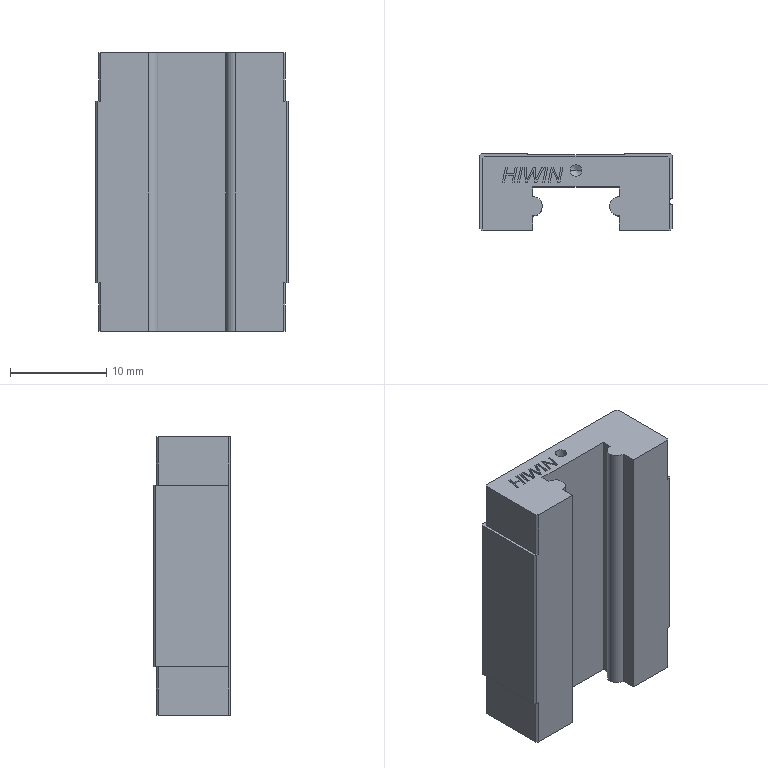Component | SolidWorks | MGN9C-10 | 1 solid | 202 faces | box 20 x 8 x 28.9 mm | volume 3299 mm3 | plane 118 | spline 55 | cylinder 17 | cone 12 | commonest cylinder face diameters 3 x8 1.2 x4 2 x3 0.6 x2